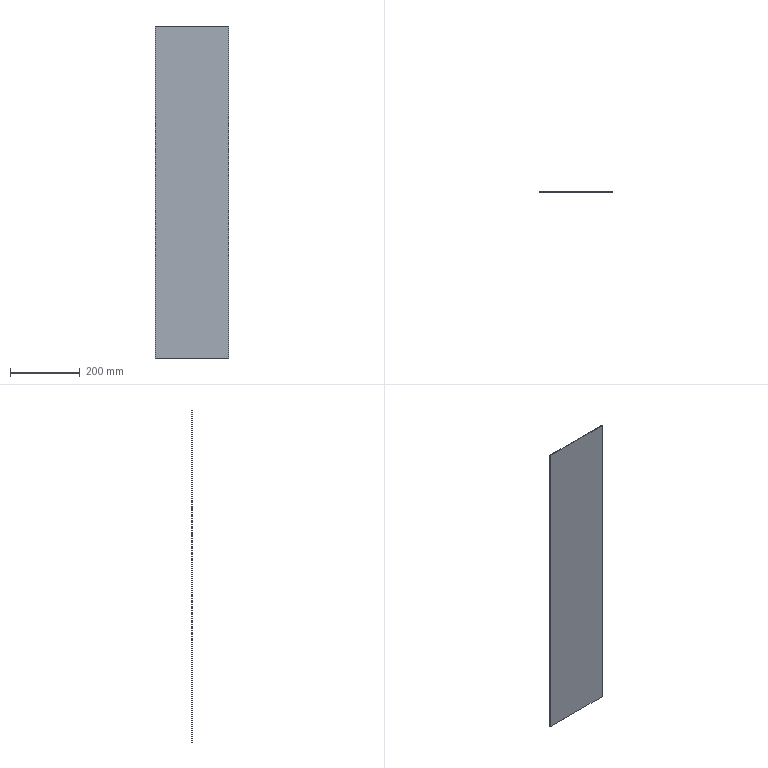Component | SolidWorks | SYM0671-81-101-1_SYM0590-81-102-3 | 1 solid | 6 faces | box 210 x 2 x 950 mm | volume 399000 mm3 | plane 6 | material Plain Carbon Steel
build123d program:
from build123d import *

# Parameters (mm, degrees)
SKETCH1_W      = 210
SKETCH1_H      = 950
EXTRUDE1_DEPTH = 2


with BuildPart() as part:
    # Sketch1 → Extrude1 (new body)
    with BuildSketch(Plane(origin=(0, 0, 0), x_dir=(1, 0, 0), z_dir=(0, 1, 0))):
        with Locations((73.603, -431.608)):
            Rectangle(SKETCH1_W, SKETCH1_H)
    extrude(amount=EXTRUDE1_DEPTH)


solid = part.part

# Placed as in the assembly
solid = solid.moved(Location((-331.351, -478.857, 83.909), (0, 0, 0)))
STEP:
#1=COLOUR_RGB('',0.7922,0.8196,0.9333);
#2=FILL_AREA_STYLE_COLOUR('',#1);
#3=FILL_AREA_STYLE('',(#2));
#4=SURFACE_STYLE_FILL_AREA(#3);
#5=SURFACE_SIDE_STYLE('',(#4));
#6=SURFACE_STYLE_USAGE(.BOTH.,#5);
#7=PRESENTATION_STYLE_ASSIGNMENT((#6));
#8=CARTESIAN_POINT('',(-14.281,-18.853,1.595));
#9=VERTEX_POINT('',#8);
#10=CARTESIAN_POINT('',(-14.281,-18.853,38.997));
#11=VERTEX_POINT('',#10);
#12=CARTESIAN_POINT('',(-14.281,-18.853,1.595));
#13=DIRECTION('',(0.,0.,1.));
#14=VECTOR('',#13,39.37);
#15=LINE('',#12,#14);
#16=EDGE_CURVE('',#9,#11,#15,.T.);
#17=ORIENTED_EDGE('',*,*,#16,.T.);
#18=CARTESIAN_POINT('',(-14.281,-18.774,38.997));
#19=VERTEX_POINT('',#18);
#20=CARTESIAN_POINT('',(-14.281,-18.774,38.997));
#21=DIRECTION('',(0.,-1.,0.));
#22=VECTOR('',#21,39.37);
#23=LINE('',#20,#22);
#24=EDGE_CURVE('',#19,#11,#23,.T.);
#25=ORIENTED_EDGE('',*,*,#24,.F.);
#26=CARTESIAN_POINT('',(-14.281,-18.774,1.595));
#27=VERTEX_POINT('',#26);
#28=CARTESIAN_POINT('',(-14.281,-18.774,1.595));
#29=DIRECTION('',(0.,0.,1.));
#30=VECTOR('',#29,39.37);
#31=LINE('',#28,#30);
#32=EDGE_CURVE('',#27,#19,#31,.T.);
#33=ORIENTED_EDGE('',*,*,#32,.F.);
#34=CARTESIAN_POINT('',(-14.281,-18.774,1.595));
#35=DIRECTION('',(0.,-1.,0.));
#36=VECTOR('',#35,39.37);
#37=LINE('',#34,#36);
#38=EDGE_CURVE('',#27,#9,#37,.T.);
#39=ORIENTED_EDGE('',*,*,#38,.T.);
#40=EDGE_LOOP('',(#17,#25,#33,#39));
#41=FACE_OUTER_BOUND('',#40,.T.);
#42=CARTESIAN_POINT('',(-14.281,-18.774,1.595));
#43=DIRECTION('',(1.,0.,-0.));
#44=DIRECTION('',(-0.,0.,-1.));
#45=AXIS2_PLACEMENT_3D('',#42,#43,#44);
#46=PLANE('',#45);
#47=ADVANCED_FACE('',(#41),#46,.F.);
#48=CARTESIAN_POINT('',(-6.014,-18.853,38.997));
#49=VERTEX_POINT('',#48);
#50=CARTESIAN_POINT('',(-14.281,-18.853,38.997));
#51=DIRECTION('',(1.,0.,0.));
#52=VECTOR('',#51,39.37);
#53=LINE('',#50,#52);
#54=EDGE_CURVE('',#11,#49,#53,.T.);
#55=ORIENTED_EDGE('',*,*,#54,.T.);
#56=CARTESIAN_POINT('',(-6.014,-18.774,38.997));
#57=VERTEX_POINT('',#56);
#58=CARTESIAN_POINT('',(-6.014,-18.774,38.997));
#59=DIRECTION('',(0.,-1.,0.));
#60=VECTOR('',#59,39.37);
#61=LINE('',#58,#60);
#62=EDGE_CURVE('',#57,#49,#61,.T.);
#63=ORIENTED_EDGE('',*,*,#62,.F.);
#64=CARTESIAN_POINT('',(-14.281,-18.774,38.997));
#65=DIRECTION('',(1.,0.,0.));
#66=VECTOR('',#65,39.37);
#67=LINE('',#64,#66);
#68=EDGE_CURVE('',#19,#57,#67,.T.);
#69=ORIENTED_EDGE('',*,*,#68,.F.);
#70=ORIENTED_EDGE('',*,*,#24,.T.);
#71=EDGE_LOOP('',(#55,#63,#69,#70));
#72=FACE_OUTER_BOUND('',#71,.T.);
#73=CARTESIAN_POINT('',(-14.281,-18.774,38.997));
#74=DIRECTION('',(0.,0.,-1.));
#75=DIRECTION('',(-1.,0.,0.));
#76=AXIS2_PLACEMENT_3D('',#73,#74,#75);
#77=PLANE('',#76);
#78=ADVANCED_FACE('',(#72),#77,.F.);
#79=CARTESIAN_POINT('',(-6.014,-18.853,1.595));
#80=VERTEX_POINT('',#79);
#81=CARTESIAN_POINT('',(-6.014,-18.853,1.595));
#82=DIRECTION('',(-0.,0.,-1.));
#83=VECTOR('',#82,39.37);
#84=LINE('',#81,#83);
#85=EDGE_CURVE('',#49,#80,#84,.T.);
#86=ORIENTED_EDGE('',*,*,#85,.T.);
#87=CARTESIAN_POINT('',(-6.014,-18.774,1.595));
#88=VERTEX_POINT('',#87);
#89=CARTESIAN_POINT('',(-6.014,-18.774,1.595));
#90=DIRECTION('',(0.,-1.,0.));
#91=VECTOR('',#90,39.37);
#92=LINE('',#89,#91);
#93=EDGE_CURVE('',#88,#80,#92,.T.);
#94=ORIENTED_EDGE('',*,*,#93,.F.);
#95=CARTESIAN_POINT('',(-6.014,-18.774,1.595));
#96=DIRECTION('',(-0.,0.,-1.));
#97=VECTOR('',#96,39.37);
#98=LINE('',#95,#97);
#99=EDGE_CURVE('',#57,#88,#98,.T.);
#100=ORIENTED_EDGE('',*,*,#99,.F.);
#101=ORIENTED_EDGE('',*,*,#62,.T.);
#102=EDGE_LOOP('',(#86,#94,#100,#101));
#103=FACE_OUTER_BOUND('',#102,.T.);
#104=CARTESIAN_POINT('',(-6.014,-18.774,1.595));
#105=DIRECTION('',(-1.,0.,0.));
#106=DIRECTION('',(0.,0.,1.));
#107=AXIS2_PLACEMENT_3D('',#104,#105,#106);
#108=PLANE('',#107);
#109=ADVANCED_FACE('',(#103),#108,.F.);
#110=CARTESIAN_POINT('',(-14.281,-18.853,1.595));
#111=DIRECTION('',(-1.,0.,0.));
#112=VECTOR('',#111,39.37);
#113=LINE('',#110,#112);
#114=EDGE_CURVE('',#80,#9,#113,.T.);
#115=ORIENTED_EDGE('',*,*,#114,.T.);
#116=ORIENTED_EDGE('',*,*,#38,.F.);
#117=CARTESIAN_POINT('',(-14.281,-18.774,1.595));
#118=DIRECTION('',(-1.,0.,0.));
#119=VECTOR('',#118,39.37);
#120=LINE('',#117,#119);
#121=EDGE_CURVE('',#88,#27,#120,.T.);
#122=ORIENTED_EDGE('',*,*,#121,.F.);
#123=ORIENTED_EDGE('',*,*,#93,.T.);
#124=EDGE_LOOP('',(#115,#116,#122,#123));
#125=FACE_OUTER_BOUND('',#124,.T.);
#126=CARTESIAN_POINT('',(-14.281,-18.774,1.595));
#127=DIRECTION('',(0.,0.,1.));
#128=DIRECTION('',(1.,0.,0.));
#129=AXIS2_PLACEMENT_3D('',#126,#127,#128);
#130=PLANE('',#129);
#131=ADVANCED_FACE('',(#125),#130,.F.);
#132=ORIENTED_EDGE('',*,*,#32,.T.);
#133=ORIENTED_EDGE('',*,*,#68,.T.);
#134=ORIENTED_EDGE('',*,*,#99,.T.);
#135=ORIENTED_EDGE('',*,*,#121,.T.);
#136=EDGE_LOOP('',(#132,#133,#134,#135));
#137=FACE_OUTER_BOUND('',#136,.T.);
#138=CARTESIAN_POINT('',(-14.281,-18.774,38.997));
#139=DIRECTION('',(0.,1.,0.));
#140=DIRECTION('',(0.,0.,1.));
#141=AXIS2_PLACEMENT_3D('',#138,#139,#140);
#142=PLANE('',#141);
#143=ADVANCED_FACE('',(#137),#142,.T.);
#144=ORIENTED_EDGE('',*,*,#16,.F.);
#145=ORIENTED_EDGE('',*,*,#114,.F.);
#146=ORIENTED_EDGE('',*,*,#85,.F.);
#147=ORIENTED_EDGE('',*,*,#54,.F.);
#148=EDGE_LOOP('',(#144,#145,#146,#147));
#149=FACE_OUTER_BOUND('',#148,.T.);
#150=CARTESIAN_POINT('',(-14.281,-18.853,38.997));
#151=DIRECTION('',(0.,1.,0.));
#152=DIRECTION('',(0.,0.,1.));
#153=AXIS2_PLACEMENT_3D('',#150,#151,#152);
#154=PLANE('',#153);
#155=ADVANCED_FACE('',(#149),#154,.F.);
#156=CLOSED_SHELL('',(#47,#78,#109,#131,#143,#155));
#157=MANIFOLD_SOLID_BREP('',#156);
#158=STYLED_ITEM('',(#7),#157);
#159=PRESENTATION_LAYER_ASSIGNMENT('','',(#158));
#160=(LENGTH_UNIT()NAMED_UNIT(*)SI_UNIT($,.METRE.));
#161=LENGTH_MEASURE_WITH_UNIT(LENGTH_MEASURE(0.0254),#160);
#162=DIMENSIONAL_EXPONENTS(1.,0.,0.,0.,0.,0.,0.);
#163=(CONVERSION_BASED_UNIT('',#161)LENGTH_UNIT()NAMED_UNIT(#162));
#164=UNCERTAINTY_MEASURE_WITH_UNIT(LENGTH_MEASURE(0.00001),#163,'','');
#165=(NAMED_UNIT(*)PLANE_ANGLE_UNIT()SI_UNIT($,.RADIAN.));
#166=(NAMED_UNIT(*)SI_UNIT($,.STERADIAN.)SOLID_ANGLE_UNIT());
#167=(GEOMETRIC_REPRESENTATION_CONTEXT(3)GLOBAL_UNCERTAINTY_ASSIGNED_CONTEXT((#164))GLOBAL_UNIT_ASSIGNED_CONTEXT((#163,#165,#166))REPRESENTATION_CONTEXT('',''));
#168=MECHANICAL_DESIGN_GEOMETRIC_PRESENTATION_REPRESENTATION('',(#158),#167);
#169=CARTESIAN_POINT('',(0.,0.,0.));
#170=DIRECTION('',(0.,0.,1.));
#171=DIRECTION('',(1.,0.,0.));
#172=AXIS2_PLACEMENT_3D('',#169,#170,#171);
#173=(LENGTH_UNIT()NAMED_UNIT(*)SI_UNIT($,.METRE.));
#174=LENGTH_MEASURE_WITH_UNIT(LENGTH_MEASURE(0.0254),#173);
#175=DIMENSIONAL_EXPONENTS(1.,0.,0.,0.,0.,0.,0.);
#176=(CONVERSION_BASED_UNIT('',#174)LENGTH_UNIT()NAMED_UNIT(#175));
#177=UNCERTAINTY_MEASURE_WITH_UNIT(LENGTH_MEASURE(0.00001),#176,'','');
#178=(NAMED_UNIT(*)PLANE_ANGLE_UNIT()SI_UNIT($,.RADIAN.));
#179=(NAMED_UNIT(*)SI_UNIT($,.STERADIAN.)SOLID_ANGLE_UNIT());
#180=(GEOMETRIC_REPRESENTATION_CONTEXT(3)GLOBAL_UNCERTAINTY_ASSIGNED_CONTEXT((#177))GLOBAL_UNIT_ASSIGNED_CONTEXT((#176,#178,#179))REPRESENTATION_CONTEXT('',''));
#181=ADVANCED_BREP_SHAPE_REPRESENTATION('',(#157,#172),#180);